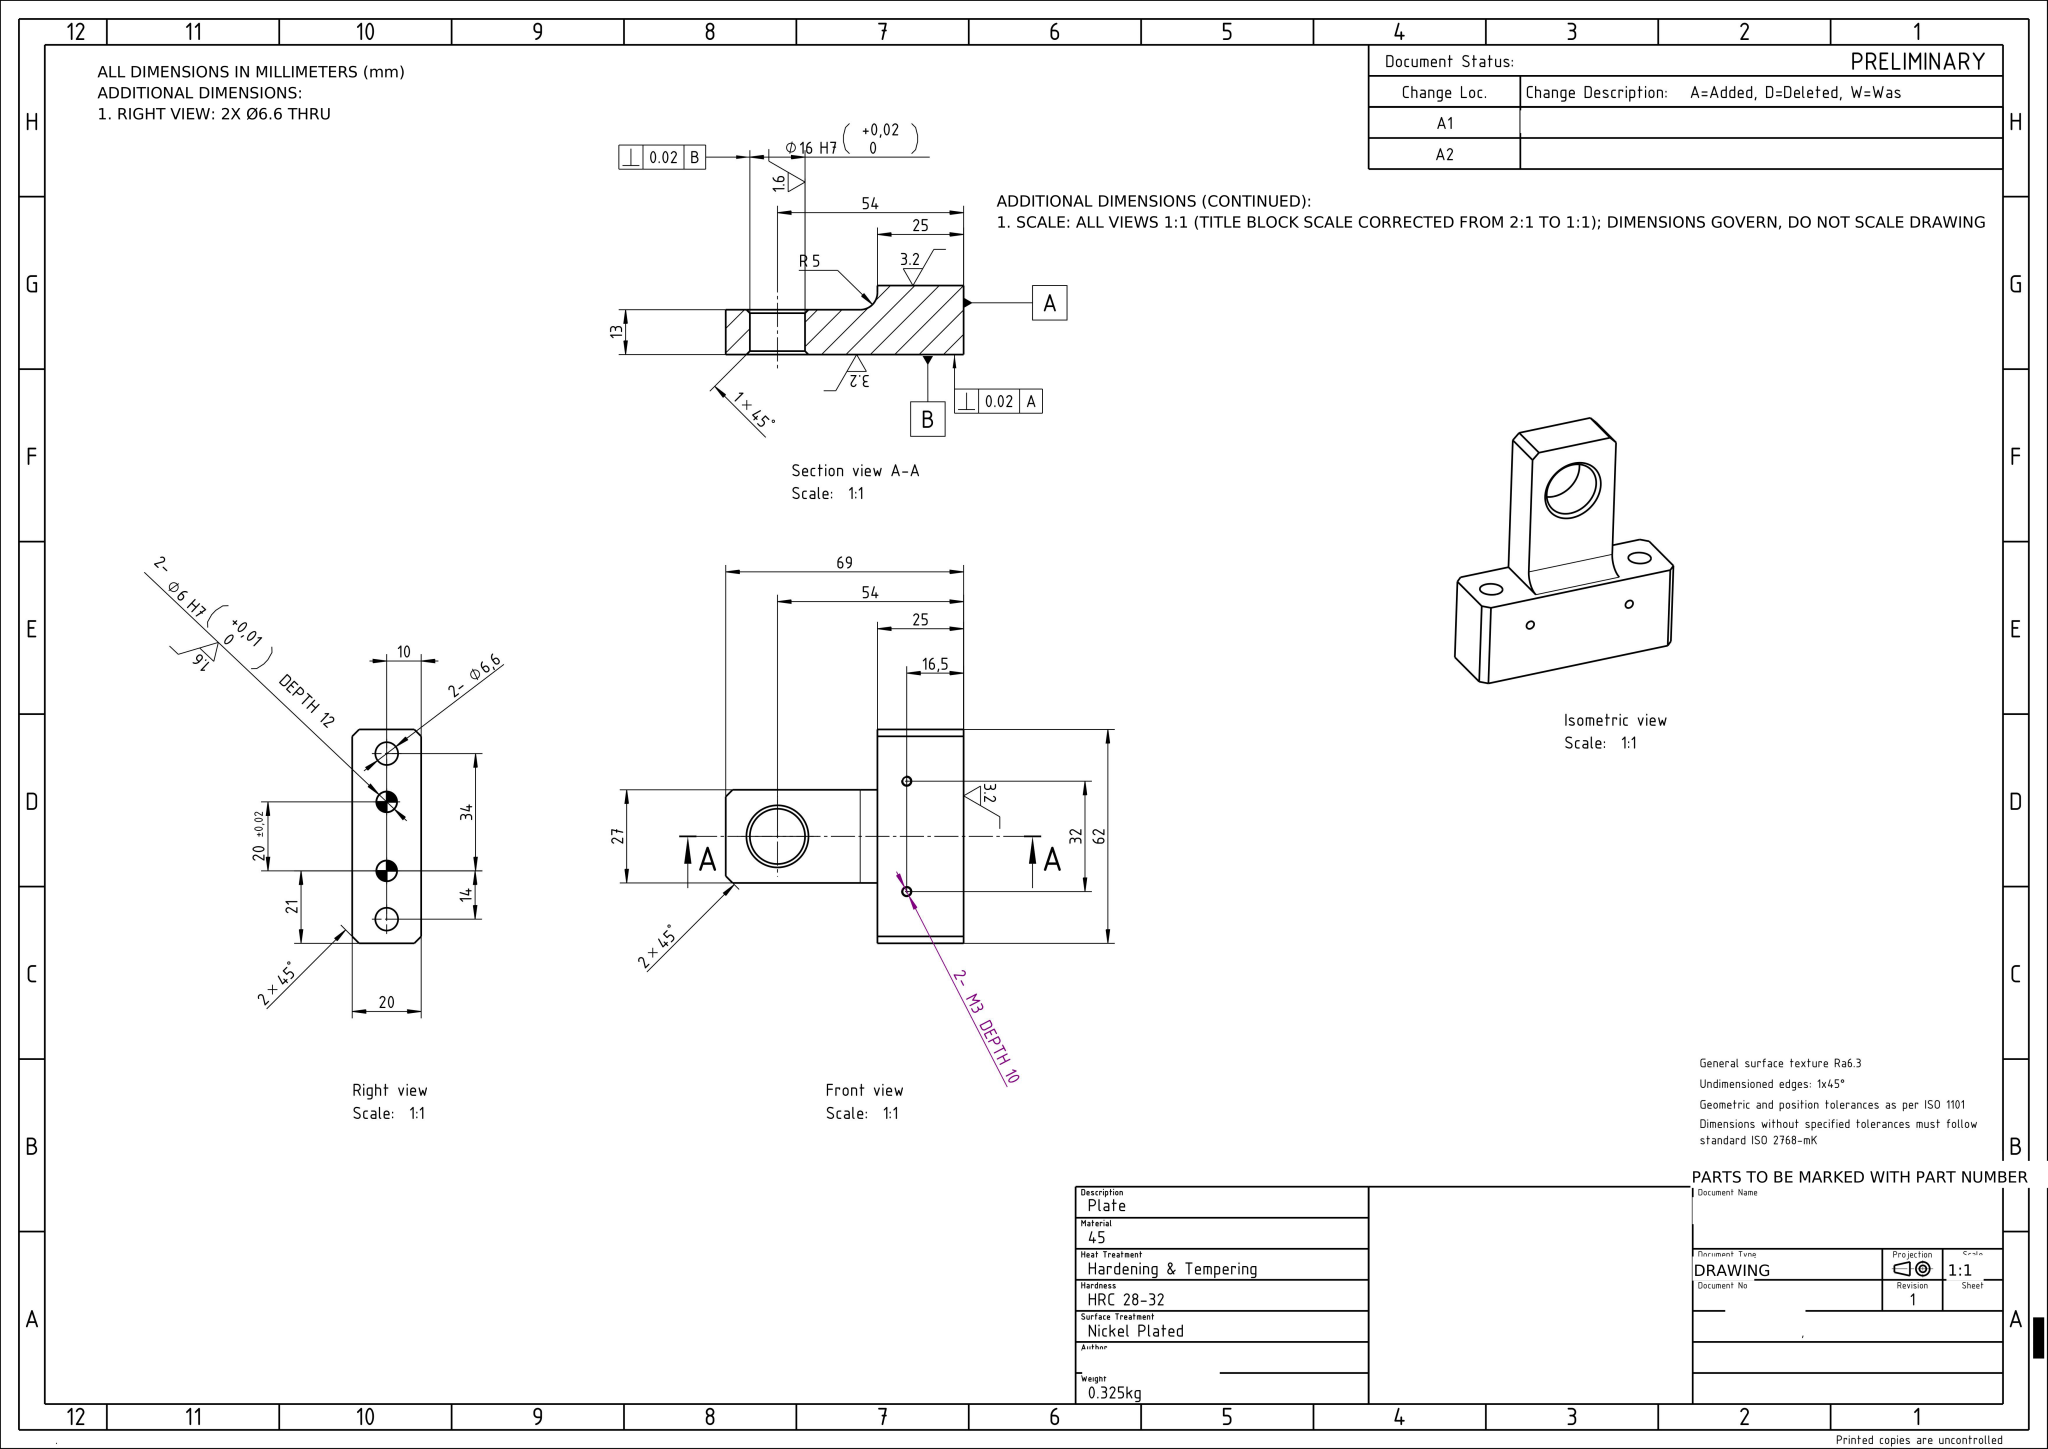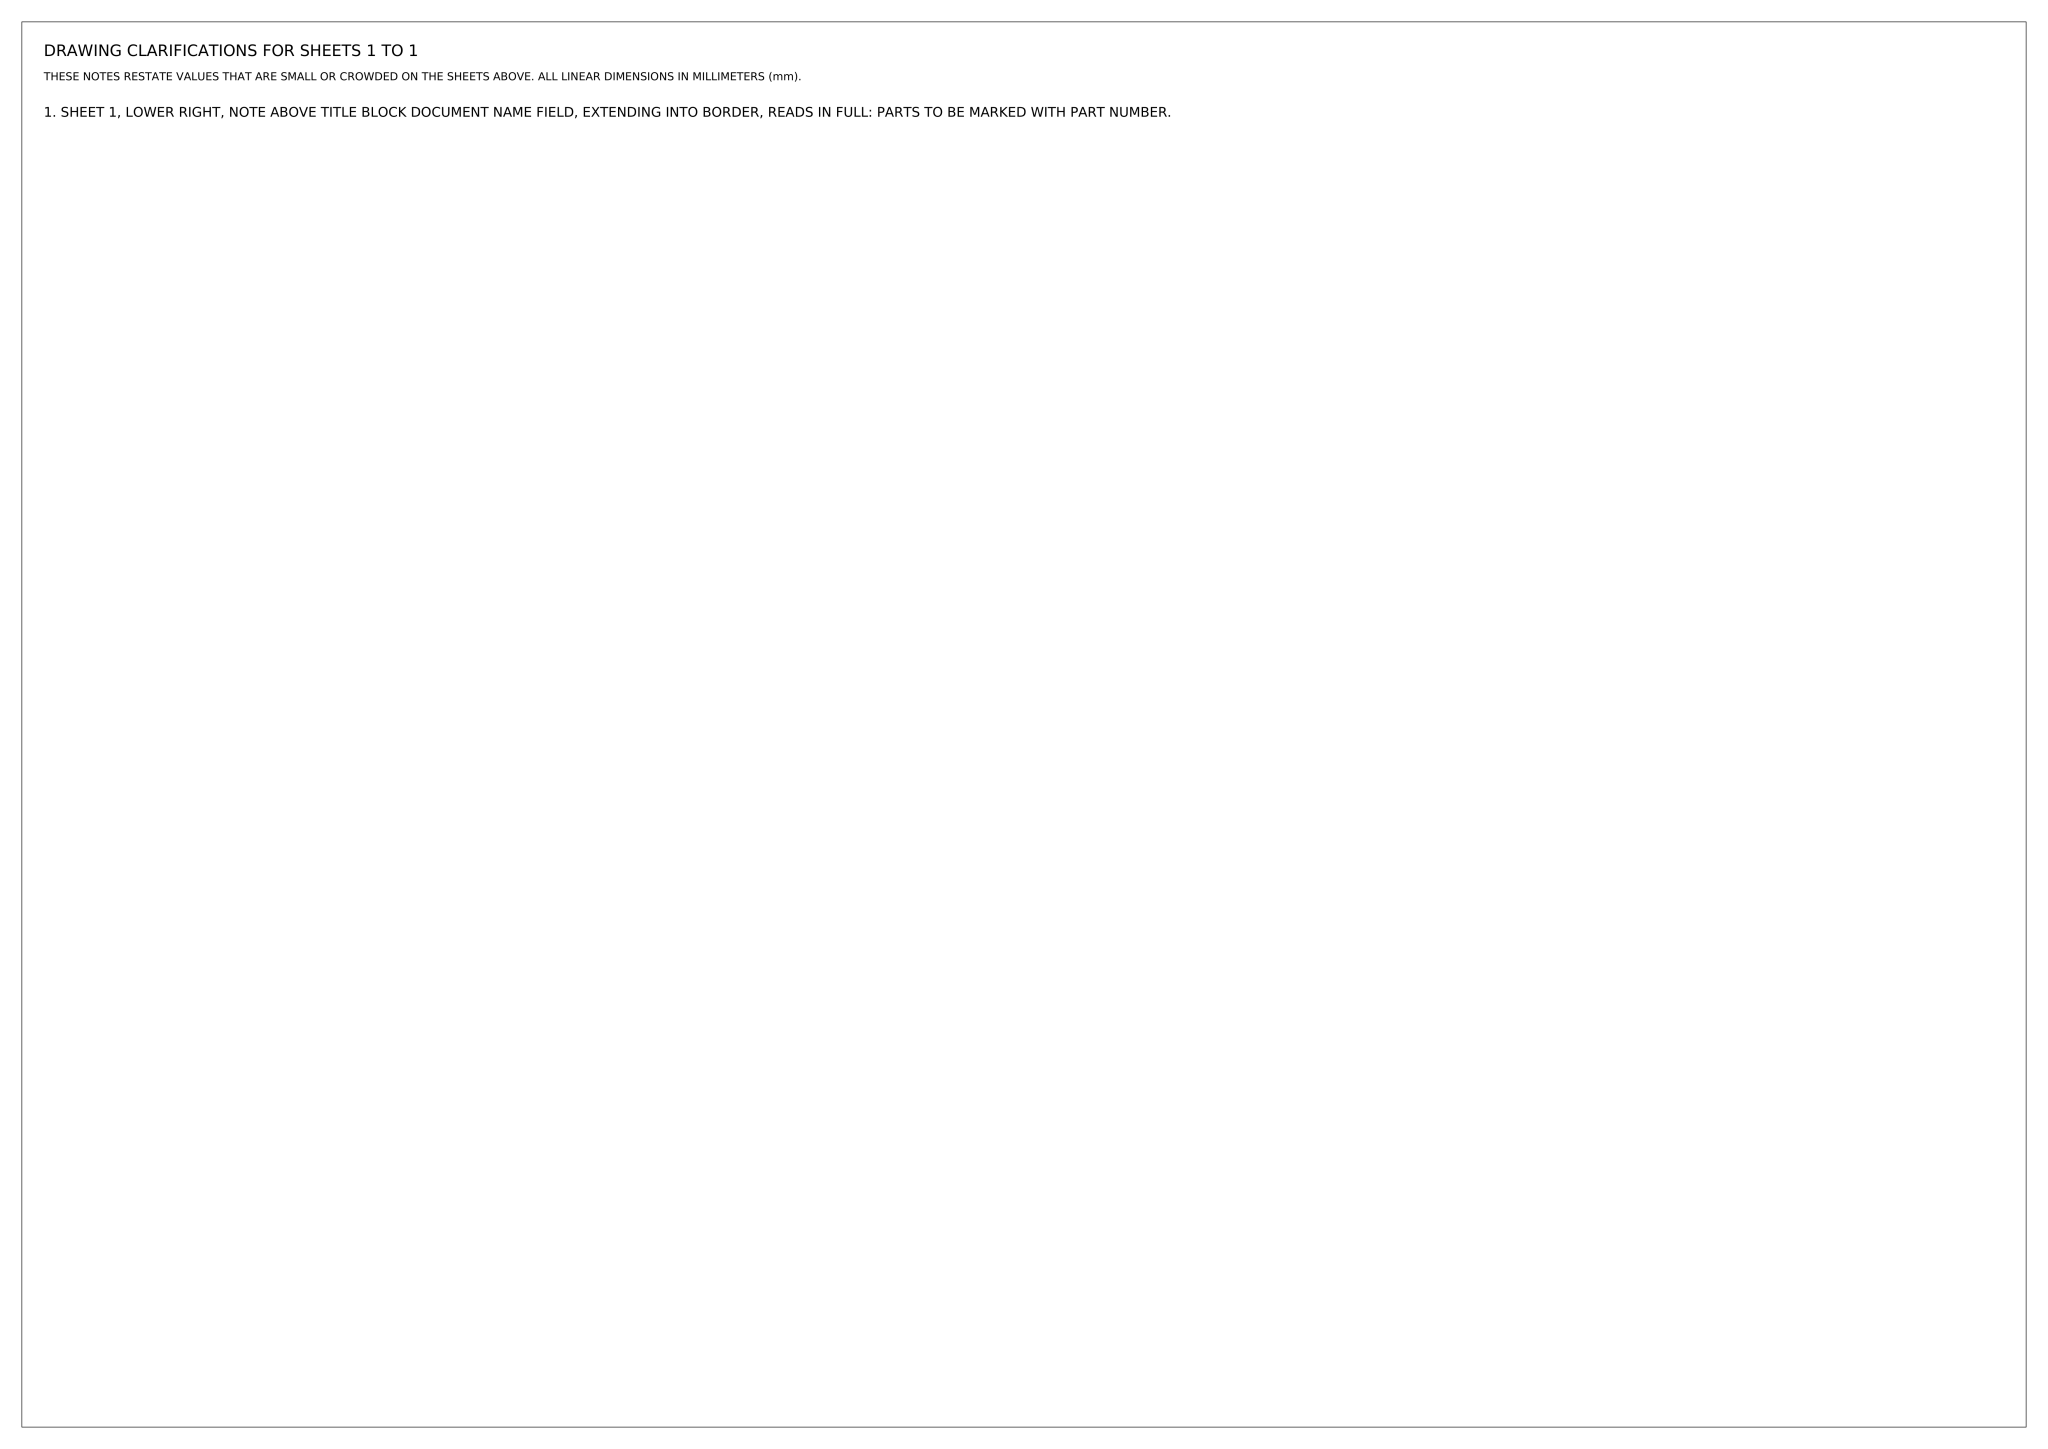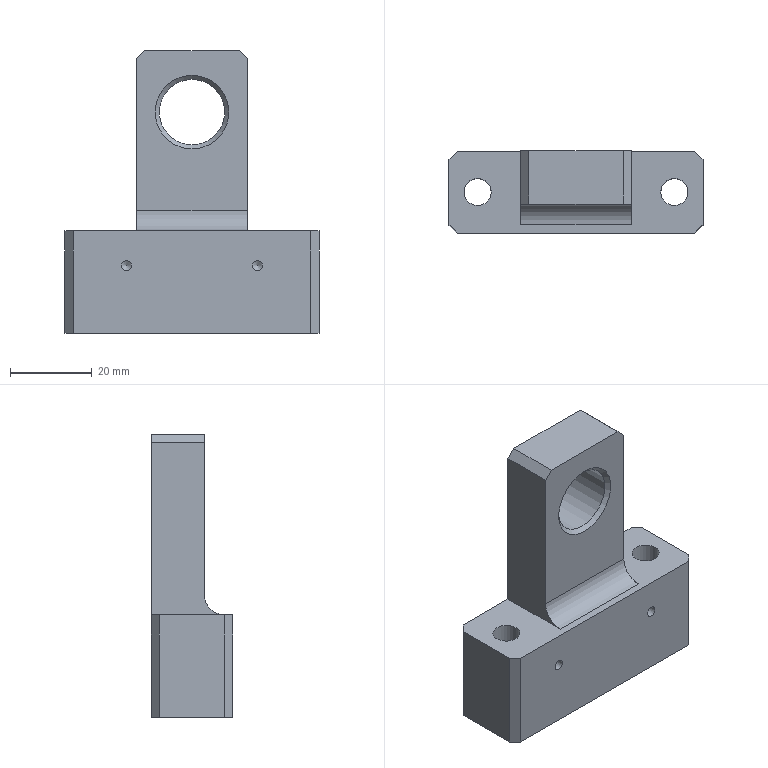Part | NX | mm | 1 solid | 30 faces | box 62 x 20 x 69 mm | volume 41127 mm3 | plane 16 | cylinder 8 | cone 6 | commonest cylinder face diameters 2.5 x2 6 x2 6.6 x2 10 x1 16 x1
STEP:
#1=CARTESIAN_POINT('',(0.,0.,0.));
#2=DIRECTION('',(0.,0.,1.));
#3=DIRECTION('',(1.,0.,0.));
#4=AXIS2_PLACEMENT_3D('',#1,#2,#3);
#5=(LENGTH_UNIT()NAMED_UNIT(*)SI_UNIT(.MILLI.,.METRE.));
#6=UNCERTAINTY_MEASURE_WITH_UNIT(LENGTH_MEASURE(0.00002),#5,'','');
#7=(NAMED_UNIT(*)PLANE_ANGLE_UNIT()SI_UNIT($,.RADIAN.));
#8=PLANE_ANGLE_MEASURE_WITH_UNIT(PLANE_ANGLE_MEASURE(0.01745),#7);
#9=DIMENSIONAL_EXPONENTS(0.,0.,0.,0.,0.,0.,0.);
#10=(CONVERSION_BASED_UNIT('',#8)NAMED_UNIT(#9)PLANE_ANGLE_UNIT());
#11=(NAMED_UNIT(*)SI_UNIT($,.STERADIAN.)SOLID_ANGLE_UNIT());
#12=(GEOMETRIC_REPRESENTATION_CONTEXT(3)GLOBAL_UNCERTAINTY_ASSIGNED_CONTEXT((#6))GLOBAL_UNIT_ASSIGNED_CONTEXT((#5,#10,#11))REPRESENTATION_CONTEXT('',''));
#13=SHAPE_REPRESENTATION('',(#4),#12);
#14=CARTESIAN_POINT('',(-31.,8.,25.));
#15=VERTEX_POINT('',#14);
#16=CARTESIAN_POINT('',(-31.,-8.,25.));
#17=VERTEX_POINT('',#16);
#18=CARTESIAN_POINT('',(-31.,10.,25.));
#19=DIRECTION('',(0.,-1.,0.));
#20=VECTOR('',#19,1.);
#21=LINE('',#18,#20);
#22=EDGE_CURVE('',#15,#17,#21,.T.);
#23=ORIENTED_EDGE('',*,*,#22,.F.);
#24=CARTESIAN_POINT('',(-31.,8.,0.));
#25=VERTEX_POINT('',#24);
#26=CARTESIAN_POINT('',(-31.,8.,25.));
#27=DIRECTION('',(0.,0.,-1.));
#28=VECTOR('',#27,1.);
#29=LINE('',#26,#28);
#30=EDGE_CURVE('',#15,#25,#29,.T.);
#31=ORIENTED_EDGE('',*,*,#30,.T.);
#32=CARTESIAN_POINT('',(-31.,-8.,0.));
#33=VERTEX_POINT('',#32);
#34=CARTESIAN_POINT('',(-31.,10.,0.));
#35=DIRECTION('',(0.,-1.,0.));
#36=VECTOR('',#35,1.);
#37=LINE('',#34,#36);
#38=EDGE_CURVE('',#25,#33,#37,.T.);
#39=ORIENTED_EDGE('',*,*,#38,.T.);
#40=CARTESIAN_POINT('',(-31.,-8.,25.));
#41=DIRECTION('',(0.,0.,1.));
#42=VECTOR('',#41,1.);
#43=LINE('',#40,#42);
#44=EDGE_CURVE('',#33,#17,#43,.T.);
#45=ORIENTED_EDGE('',*,*,#44,.T.);
#46=EDGE_LOOP('',(#23,#31,#39,#45));
#47=FACE_OUTER_BOUND('',#46,.T.);
#48=CARTESIAN_POINT('',(-31.,10.,25.));
#49=DIRECTION('',(1.,0.,0.));
#50=DIRECTION('',(-0.,1.,0.));
#51=AXIS2_PLACEMENT_3D('',#48,#49,#50);
#52=PLANE('',#51);
#53=ADVANCED_FACE('',(#47),#52,.F.);
#54=CARTESIAN_POINT('',(16.,-10.,17.75));
#55=VERTEX_POINT('',#54);
#56=CARTESIAN_POINT('',(16.,-10.,16.5));
#57=DIRECTION('',(0.,1.,0.));
#58=DIRECTION('',(0.,0.,1.));
#59=AXIS2_PLACEMENT_3D('',#56,#57,#58);
#60=CIRCLE('',#59,1.25);
#61=EDGE_CURVE('',#55,#55,#60,.T.);
#62=ORIENTED_EDGE('',*,*,#61,.T.);
#63=EDGE_LOOP('',(#62));
#64=FACE_BOUND('',#63,.T.);
#65=CARTESIAN_POINT('',(-16.,-10.,17.75));
#66=VERTEX_POINT('',#65);
#67=CARTESIAN_POINT('',(-16.,-10.,16.5));
#68=DIRECTION('',(0.,1.,0.));
#69=DIRECTION('',(0.,0.,1.));
#70=AXIS2_PLACEMENT_3D('',#67,#68,#69);
#71=CIRCLE('',#70,1.25);
#72=EDGE_CURVE('',#66,#66,#71,.T.);
#73=ORIENTED_EDGE('',*,*,#72,.T.);
#74=EDGE_LOOP('',(#73));
#75=FACE_BOUND('',#74,.T.);
#76=CARTESIAN_POINT('',(-29.,-10.,0.));
#77=VERTEX_POINT('',#76);
#78=CARTESIAN_POINT('',(29.,-10.,0.));
#79=VERTEX_POINT('',#78);
#80=CARTESIAN_POINT('',(-31.,-10.,0.));
#81=DIRECTION('',(1.,0.,0.));
#82=VECTOR('',#81,1.);
#83=LINE('',#80,#82);
#84=EDGE_CURVE('',#77,#79,#83,.T.);
#85=ORIENTED_EDGE('',*,*,#84,.T.);
#86=CARTESIAN_POINT('',(29.,-10.,25.));
#87=VERTEX_POINT('',#86);
#88=CARTESIAN_POINT('',(29.,-10.,25.));
#89=DIRECTION('',(0.,0.,1.));
#90=VECTOR('',#89,1.);
#91=LINE('',#88,#90);
#92=EDGE_CURVE('',#79,#87,#91,.T.);
#93=ORIENTED_EDGE('',*,*,#92,.T.);
#94=CARTESIAN_POINT('',(-29.,-10.,25.));
#95=VERTEX_POINT('',#94);
#96=CARTESIAN_POINT('',(-31.,-10.,25.));
#97=DIRECTION('',(1.,0.,0.));
#98=VECTOR('',#97,1.);
#99=LINE('',#96,#98);
#100=EDGE_CURVE('',#95,#87,#99,.T.);
#101=ORIENTED_EDGE('',*,*,#100,.F.);
#102=CARTESIAN_POINT('',(-29.,-10.,25.));
#103=DIRECTION('',(0.,0.,-1.));
#104=VECTOR('',#103,1.);
#105=LINE('',#102,#104);
#106=EDGE_CURVE('',#95,#77,#105,.T.);
#107=ORIENTED_EDGE('',*,*,#106,.T.);
#108=EDGE_LOOP('',(#85,#93,#101,#107));
#109=FACE_BOUND('',#108,.T.);
#110=CARTESIAN_POINT('',(-31.,-10.,25.));
#111=DIRECTION('',(0.,1.,0.));
#112=DIRECTION('',(0.,0.,1.));
#113=AXIS2_PLACEMENT_3D('',#110,#111,#112);
#114=PLANE('',#113);
#115=ADVANCED_FACE('',(#64,#75,#109),#114,.F.);
#116=CARTESIAN_POINT('',(31.,-8.,25.));
#117=VERTEX_POINT('',#116);
#118=CARTESIAN_POINT('',(31.,8.,25.));
#119=VERTEX_POINT('',#118);
#120=CARTESIAN_POINT('',(31.,-10.,25.));
#121=DIRECTION('',(-0.,1.,0.));
#122=VECTOR('',#121,1.);
#123=LINE('',#120,#122);
#124=EDGE_CURVE('',#117,#119,#123,.T.);
#125=ORIENTED_EDGE('',*,*,#124,.F.);
#126=CARTESIAN_POINT('',(31.,-8.,0.));
#127=VERTEX_POINT('',#126);
#128=CARTESIAN_POINT('',(31.,-8.,25.));
#129=DIRECTION('',(0.,0.,-1.));
#130=VECTOR('',#129,1.);
#131=LINE('',#128,#130);
#132=EDGE_CURVE('',#117,#127,#131,.T.);
#133=ORIENTED_EDGE('',*,*,#132,.T.);
#134=CARTESIAN_POINT('',(31.,8.,0.));
#135=VERTEX_POINT('',#134);
#136=CARTESIAN_POINT('',(31.,-10.,0.));
#137=DIRECTION('',(-0.,1.,0.));
#138=VECTOR('',#137,1.);
#139=LINE('',#136,#138);
#140=EDGE_CURVE('',#127,#135,#139,.T.);
#141=ORIENTED_EDGE('',*,*,#140,.T.);
#142=CARTESIAN_POINT('',(31.,8.,25.));
#143=DIRECTION('',(0.,0.,1.));
#144=VECTOR('',#143,1.);
#145=LINE('',#142,#144);
#146=EDGE_CURVE('',#135,#119,#145,.T.);
#147=ORIENTED_EDGE('',*,*,#146,.T.);
#148=EDGE_LOOP('',(#125,#133,#141,#147));
#149=FACE_OUTER_BOUND('',#148,.T.);
#150=CARTESIAN_POINT('',(31.,-10.,25.));
#151=DIRECTION('',(-1.,-0.,0.));
#152=DIRECTION('',(0.,-1.,0.));
#153=AXIS2_PLACEMENT_3D('',#150,#151,#152);
#154=PLANE('',#153);
#155=ADVANCED_FACE('',(#149),#154,.F.);
#156=CARTESIAN_POINT('',(0.,10.,45.));
#157=VERTEX_POINT('',#156);
#158=CARTESIAN_POINT('',(0.,10.,54.));
#159=DIRECTION('',(0.,-1.,0.));
#160=DIRECTION('',(0.,0.,-1.));
#161=AXIS2_PLACEMENT_3D('',#158,#159,#160);
#162=CIRCLE('',#161,9.);
#163=EDGE_CURVE('',#157,#157,#162,.T.);
#164=ORIENTED_EDGE('',*,*,#163,.T.);
#165=EDGE_LOOP('',(#164));
#166=FACE_BOUND('',#165,.T.);
#167=CARTESIAN_POINT('',(29.,10.,25.));
#168=VERTEX_POINT('',#167);
#169=CARTESIAN_POINT('',(13.5,10.,25.));
#170=VERTEX_POINT('',#169);
#171=CARTESIAN_POINT('',(31.,10.,25.));
#172=DIRECTION('',(-1.,0.,0.));
#173=VECTOR('',#172,1.);
#174=LINE('',#171,#173);
#175=EDGE_CURVE('',#168,#170,#174,.T.);
#176=ORIENTED_EDGE('',*,*,#175,.F.);
#177=CARTESIAN_POINT('',(29.,10.,0.));
#178=VERTEX_POINT('',#177);
#179=CARTESIAN_POINT('',(29.,10.,25.));
#180=DIRECTION('',(0.,0.,-1.));
#181=VECTOR('',#180,1.);
#182=LINE('',#179,#181);
#183=EDGE_CURVE('',#168,#178,#182,.T.);
#184=ORIENTED_EDGE('',*,*,#183,.T.);
#185=CARTESIAN_POINT('',(-29.,10.,0.));
#186=VERTEX_POINT('',#185);
#187=CARTESIAN_POINT('',(31.,10.,0.));
#188=DIRECTION('',(-1.,0.,0.));
#189=VECTOR('',#188,1.);
#190=LINE('',#187,#189);
#191=EDGE_CURVE('',#178,#186,#190,.T.);
#192=ORIENTED_EDGE('',*,*,#191,.T.);
#193=CARTESIAN_POINT('',(-29.,10.,25.));
#194=VERTEX_POINT('',#193);
#195=CARTESIAN_POINT('',(-29.,10.,25.));
#196=DIRECTION('',(0.,0.,1.));
#197=VECTOR('',#196,1.);
#198=LINE('',#195,#197);
#199=EDGE_CURVE('',#186,#194,#198,.T.);
#200=ORIENTED_EDGE('',*,*,#199,.T.);
#201=CARTESIAN_POINT('',(-13.5,10.,25.));
#202=VERTEX_POINT('',#201);
#203=CARTESIAN_POINT('',(31.,10.,25.));
#204=DIRECTION('',(-1.,0.,0.));
#205=VECTOR('',#204,1.);
#206=LINE('',#203,#205);
#207=EDGE_CURVE('',#202,#194,#206,.T.);
#208=ORIENTED_EDGE('',*,*,#207,.F.);
#209=CARTESIAN_POINT('',(-13.5,10.,67.));
#210=VERTEX_POINT('',#209);
#211=CARTESIAN_POINT('',(-13.5,10.,25.));
#212=DIRECTION('',(0.,0.,1.));
#213=VECTOR('',#212,1.);
#214=LINE('',#211,#213);
#215=EDGE_CURVE('',#202,#210,#214,.T.);
#216=ORIENTED_EDGE('',*,*,#215,.T.);
#217=CARTESIAN_POINT('',(-11.5,10.,69.));
#218=VERTEX_POINT('',#217);
#219=CARTESIAN_POINT('',(-13.5,10.,67.));
#220=DIRECTION('',(0.7071,0.,0.7071));
#221=VECTOR('',#220,1.);
#222=LINE('',#219,#221);
#223=EDGE_CURVE('',#210,#218,#222,.T.);
#224=ORIENTED_EDGE('',*,*,#223,.T.);
#225=CARTESIAN_POINT('',(11.5,10.,69.));
#226=VERTEX_POINT('',#225);
#227=CARTESIAN_POINT('',(-13.5,10.,69.));
#228=DIRECTION('',(1.,0.,0.));
#229=VECTOR('',#228,1.);
#230=LINE('',#227,#229);
#231=EDGE_CURVE('',#218,#226,#230,.T.);
#232=ORIENTED_EDGE('',*,*,#231,.T.);
#233=CARTESIAN_POINT('',(13.5,10.,67.));
#234=VERTEX_POINT('',#233);
#235=CARTESIAN_POINT('',(11.5,10.,69.));
#236=DIRECTION('',(0.7071,0.,-0.7071));
#237=VECTOR('',#236,1.);
#238=LINE('',#235,#237);
#239=EDGE_CURVE('',#226,#234,#238,.T.);
#240=ORIENTED_EDGE('',*,*,#239,.T.);
#241=CARTESIAN_POINT('',(13.5,10.,69.));
#242=DIRECTION('',(0.,0.,-1.));
#243=VECTOR('',#242,1.);
#244=LINE('',#241,#243);
#245=EDGE_CURVE('',#234,#170,#244,.T.);
#246=ORIENTED_EDGE('',*,*,#245,.T.);
#247=EDGE_LOOP('',(#176,#184,#192,#200,#208,#216,#224,#232,#240,#246));
#248=FACE_BOUND('',#247,.T.);
#249=CARTESIAN_POINT('',(31.,10.,25.));
#250=DIRECTION('',(0.,-1.,0.));
#251=DIRECTION('',(0.,0.,-1.));
#252=AXIS2_PLACEMENT_3D('',#249,#250,#251);
#253=PLANE('',#252);
#254=ADVANCED_FACE('',(#166,#248),#253,.F.);
#255=CARTESIAN_POINT('',(27.3,0.,25.));
#256=VERTEX_POINT('',#255);
#257=CARTESIAN_POINT('',(24.,0.,25.));
#258=DIRECTION('',(0.,0.,1.));
#259=DIRECTION('',(1.,0.,0.));
#260=AXIS2_PLACEMENT_3D('',#257,#258,#259);
#261=CIRCLE('',#260,3.3);
#262=EDGE_CURVE('',#256,#256,#261,.T.);
#263=ORIENTED_EDGE('',*,*,#262,.F.);
#264=EDGE_LOOP('',(#263));
#265=FACE_BOUND('',#264,.T.);
#266=CARTESIAN_POINT('',(-20.7,0.,25.));
#267=VERTEX_POINT('',#266);
#268=CARTESIAN_POINT('',(-24.,0.,25.));
#269=DIRECTION('',(0.,0.,1.));
#270=DIRECTION('',(1.,0.,0.));
#271=AXIS2_PLACEMENT_3D('',#268,#269,#270);
#272=CIRCLE('',#271,3.3);
#273=EDGE_CURVE('',#267,#267,#272,.T.);
#274=ORIENTED_EDGE('',*,*,#273,.F.);
#275=EDGE_LOOP('',(#274));
#276=FACE_BOUND('',#275,.T.);
#277=ORIENTED_EDGE('',*,*,#100,.T.);
#278=CARTESIAN_POINT('',(19.5,-19.5,25.));
#279=DIRECTION('',(0.7071,0.7071,0.));
#280=VECTOR('',#279,1.);
#281=LINE('',#278,#280);
#282=EDGE_CURVE('',#87,#117,#281,.T.);
#283=ORIENTED_EDGE('',*,*,#282,.T.);
#284=ORIENTED_EDGE('',*,*,#124,.T.);
#285=CARTESIAN_POINT('',(19.5,19.5,25.));
#286=DIRECTION('',(-0.7071,0.7071,0.));
#287=VECTOR('',#286,1.);
#288=LINE('',#285,#287);
#289=EDGE_CURVE('',#119,#168,#288,.T.);
#290=ORIENTED_EDGE('',*,*,#289,.T.);
#291=ORIENTED_EDGE('',*,*,#175,.T.);
#292=CARTESIAN_POINT('',(13.5,-8.,25.));
#293=VERTEX_POINT('',#292);
#294=CARTESIAN_POINT('',(13.5,-3.,25.));
#295=DIRECTION('',(0.,1.,0.));
#296=VECTOR('',#295,1.);
#297=LINE('',#294,#296);
#298=EDGE_CURVE('',#293,#170,#297,.T.);
#299=ORIENTED_EDGE('',*,*,#298,.F.);
#300=CARTESIAN_POINT('',(-13.5,-8.,25.));
#301=VERTEX_POINT('',#300);
#302=CARTESIAN_POINT('',(0.,-8.,25.));
#303=DIRECTION('',(-1.,0.,0.));
#304=VECTOR('',#303,1.);
#305=LINE('',#302,#304);
#306=EDGE_CURVE('',#293,#301,#305,.T.);
#307=ORIENTED_EDGE('',*,*,#306,.T.);
#308=CARTESIAN_POINT('',(-13.5,-3.,25.));
#309=DIRECTION('',(0.,1.,0.));
#310=VECTOR('',#309,1.);
#311=LINE('',#308,#310);
#312=EDGE_CURVE('',#301,#202,#311,.T.);
#313=ORIENTED_EDGE('',*,*,#312,.T.);
#314=ORIENTED_EDGE('',*,*,#207,.T.);
#315=CARTESIAN_POINT('',(-19.5,19.5,25.));
#316=DIRECTION('',(-0.7071,-0.7071,0.));
#317=VECTOR('',#316,1.);
#318=LINE('',#315,#317);
#319=EDGE_CURVE('',#194,#15,#318,.T.);
#320=ORIENTED_EDGE('',*,*,#319,.T.);
#321=ORIENTED_EDGE('',*,*,#22,.T.);
#322=CARTESIAN_POINT('',(-19.5,-19.5,25.));
#323=DIRECTION('',(0.7071,-0.7071,0.));
#324=VECTOR('',#323,1.);
#325=LINE('',#322,#324);
#326=EDGE_CURVE('',#17,#95,#325,.T.);
#327=ORIENTED_EDGE('',*,*,#326,.T.);
#328=EDGE_LOOP('',(#277,#283,#284,#290,#291,#299,#307,#313,#314,#320,#321,#327));
#329=FACE_BOUND('',#328,.T.);
#330=CARTESIAN_POINT('',(0.,0.,25.));
#331=DIRECTION('',(0.,0.,1.));
#332=DIRECTION('',(1.,0.,0.));
#333=AXIS2_PLACEMENT_3D('',#330,#331,#332);
#334=PLANE('',#333);
#335=ADVANCED_FACE('',(#265,#276,#329),#334,.T.);
#336=CARTESIAN_POINT('',(27.3,0.,0.));
#337=VERTEX_POINT('',#336);
#338=CARTESIAN_POINT('',(24.,0.,0.));
#339=DIRECTION('',(0.,0.,1.));
#340=DIRECTION('',(1.,0.,0.));
#341=AXIS2_PLACEMENT_3D('',#338,#339,#340);
#342=CIRCLE('',#341,3.3);
#343=EDGE_CURVE('',#337,#337,#342,.T.);
#344=ORIENTED_EDGE('',*,*,#343,.T.);
#345=EDGE_LOOP('',(#344));
#346=FACE_BOUND('',#345,.T.);
#347=CARTESIAN_POINT('',(-20.7,0.,0.));
#348=VERTEX_POINT('',#347);
#349=CARTESIAN_POINT('',(-24.,0.,0.));
#350=DIRECTION('',(0.,0.,1.));
#351=DIRECTION('',(1.,0.,0.));
#352=AXIS2_PLACEMENT_3D('',#349,#350,#351);
#353=CIRCLE('',#352,3.3);
#354=EDGE_CURVE('',#348,#348,#353,.T.);
#355=ORIENTED_EDGE('',*,*,#354,.T.);
#356=EDGE_LOOP('',(#355));
#357=FACE_BOUND('',#356,.T.);
#358=CARTESIAN_POINT('',(13.,0.,0.));
#359=VERTEX_POINT('',#358);
#360=CARTESIAN_POINT('',(10.,0.,0.));
#361=DIRECTION('',(0.,0.,1.));
#362=DIRECTION('',(1.,0.,0.));
#363=AXIS2_PLACEMENT_3D('',#360,#361,#362);
#364=CIRCLE('',#363,3.);
#365=EDGE_CURVE('',#359,#359,#364,.T.);
#366=ORIENTED_EDGE('',*,*,#365,.T.);
#367=EDGE_LOOP('',(#366));
#368=FACE_BOUND('',#367,.T.);
#369=CARTESIAN_POINT('',(-7.,0.,0.));
#370=VERTEX_POINT('',#369);
#371=CARTESIAN_POINT('',(-10.,0.,0.));
#372=DIRECTION('',(0.,0.,1.));
#373=DIRECTION('',(1.,0.,0.));
#374=AXIS2_PLACEMENT_3D('',#371,#372,#373);
#375=CIRCLE('',#374,3.);
#376=EDGE_CURVE('',#370,#370,#375,.T.);
#377=ORIENTED_EDGE('',*,*,#376,.T.);
#378=EDGE_LOOP('',(#377));
#379=FACE_BOUND('',#378,.T.);
#380=ORIENTED_EDGE('',*,*,#140,.F.);
#381=CARTESIAN_POINT('',(31.,-8.,0.));
#382=DIRECTION('',(-0.7071,-0.7071,0.));
#383=VECTOR('',#382,1.);
#384=LINE('',#381,#383);
#385=EDGE_CURVE('',#127,#79,#384,.T.);
#386=ORIENTED_EDGE('',*,*,#385,.T.);
#387=ORIENTED_EDGE('',*,*,#84,.F.);
#388=CARTESIAN_POINT('',(-29.,-10.,0.));
#389=DIRECTION('',(-0.7071,0.7071,0.));
#390=VECTOR('',#389,1.);
#391=LINE('',#388,#390);
#392=EDGE_CURVE('',#77,#33,#391,.T.);
#393=ORIENTED_EDGE('',*,*,#392,.T.);
#394=ORIENTED_EDGE('',*,*,#38,.F.);
#395=CARTESIAN_POINT('',(-31.,8.,0.));
#396=DIRECTION('',(0.7071,0.7071,0.));
#397=VECTOR('',#396,1.);
#398=LINE('',#395,#397);
#399=EDGE_CURVE('',#25,#186,#398,.T.);
#400=ORIENTED_EDGE('',*,*,#399,.T.);
#401=ORIENTED_EDGE('',*,*,#191,.F.);
#402=CARTESIAN_POINT('',(29.,10.,0.));
#403=DIRECTION('',(0.7071,-0.7071,0.));
#404=VECTOR('',#403,1.);
#405=LINE('',#402,#404);
#406=EDGE_CURVE('',#178,#135,#405,.T.);
#407=ORIENTED_EDGE('',*,*,#406,.T.);
#408=EDGE_LOOP('',(#380,#386,#387,#393,#394,#400,#401,#407));
#409=FACE_BOUND('',#408,.T.);
#410=CARTESIAN_POINT('',(0.,0.,0.));
#411=DIRECTION('',(0.,0.,1.));
#412=DIRECTION('',(1.,0.,0.));
#413=AXIS2_PLACEMENT_3D('',#410,#411,#412);
#414=PLANE('',#413);
#415=ADVANCED_FACE('',(#346,#357,#368,#379,#409),#414,.F.);
#416=CARTESIAN_POINT('',(-13.5,-3.,30.));
#417=VERTEX_POINT('',#416);
#418=CARTESIAN_POINT('',(-13.5,-3.,67.));
#419=VERTEX_POINT('',#418);
#420=CARTESIAN_POINT('',(-13.5,-3.,25.));
#421=DIRECTION('',(0.,0.,1.));
#422=VECTOR('',#421,1.);
#423=LINE('',#420,#422);
#424=EDGE_CURVE('',#417,#419,#423,.T.);
#425=ORIENTED_EDGE('',*,*,#424,.T.);
#426=CARTESIAN_POINT('',(-13.5,-3.,67.));
#427=DIRECTION('',(0.,1.,0.));
#428=VECTOR('',#427,1.);
#429=LINE('',#426,#428);
#430=EDGE_CURVE('',#419,#210,#429,.T.);
#431=ORIENTED_EDGE('',*,*,#430,.T.);
#432=ORIENTED_EDGE('',*,*,#215,.F.);
#433=ORIENTED_EDGE('',*,*,#312,.F.);
#434=CARTESIAN_POINT('',(-13.5,-8.,30.));
#435=DIRECTION('',(1.,0.,0.));
#436=DIRECTION('',(0.,0.,1.));
#437=AXIS2_PLACEMENT_3D('',#434,#435,#436);
#438=CIRCLE('',#437,5.);
#439=EDGE_CURVE('',#301,#417,#438,.T.);
#440=ORIENTED_EDGE('',*,*,#439,.T.);
#441=EDGE_LOOP('',(#425,#431,#432,#433,#440));
#442=FACE_OUTER_BOUND('',#441,.T.);
#443=CARTESIAN_POINT('',(-13.5,-3.,25.));
#444=DIRECTION('',(-1.,0.,0.));
#445=DIRECTION('',(0.,0.,1.));
#446=AXIS2_PLACEMENT_3D('',#443,#444,#445);
#447=PLANE('',#446);
#448=ADVANCED_FACE('',(#442),#447,.T.);
#449=ORIENTED_EDGE('',*,*,#231,.F.);
#450=CARTESIAN_POINT('',(-11.5,-3.,69.));
#451=VERTEX_POINT('',#450);
#452=CARTESIAN_POINT('',(-11.5,-3.,69.));
#453=DIRECTION('',(0.,-1.,0.));
#454=VECTOR('',#453,1.);
#455=LINE('',#452,#454);
#456=EDGE_CURVE('',#218,#451,#455,.T.);
#457=ORIENTED_EDGE('',*,*,#456,.T.);
#458=CARTESIAN_POINT('',(11.5,-3.,69.));
#459=VERTEX_POINT('',#458);
#460=CARTESIAN_POINT('',(-13.5,-3.,69.));
#461=DIRECTION('',(1.,0.,0.));
#462=VECTOR('',#461,1.);
#463=LINE('',#460,#462);
#464=EDGE_CURVE('',#451,#459,#463,.T.);
#465=ORIENTED_EDGE('',*,*,#464,.T.);
#466=CARTESIAN_POINT('',(11.5,-3.,69.));
#467=DIRECTION('',(0.,1.,0.));
#468=VECTOR('',#467,1.);
#469=LINE('',#466,#468);
#470=EDGE_CURVE('',#459,#226,#469,.T.);
#471=ORIENTED_EDGE('',*,*,#470,.T.);
#472=EDGE_LOOP('',(#449,#457,#465,#471));
#473=FACE_OUTER_BOUND('',#472,.T.);
#474=CARTESIAN_POINT('',(-13.5,-3.,69.));
#475=DIRECTION('',(0.,0.,1.));
#476=DIRECTION('',(1.,0.,0.));
#477=AXIS2_PLACEMENT_3D('',#474,#475,#476);
#478=PLANE('',#477);
#479=ADVANCED_FACE('',(#473),#478,.T.);
#480=ORIENTED_EDGE('',*,*,#245,.F.);
#481=CARTESIAN_POINT('',(13.5,-3.,67.));
#482=VERTEX_POINT('',#481);
#483=CARTESIAN_POINT('',(13.5,-3.,67.));
#484=DIRECTION('',(0.,-1.,0.));
#485=VECTOR('',#484,1.);
#486=LINE('',#483,#485);
#487=EDGE_CURVE('',#234,#482,#486,.T.);
#488=ORIENTED_EDGE('',*,*,#487,.T.);
#489=CARTESIAN_POINT('',(13.5,-3.,30.));
#490=VERTEX_POINT('',#489);
#491=CARTESIAN_POINT('',(13.5,-3.,69.));
#492=DIRECTION('',(0.,0.,-1.));
#493=VECTOR('',#492,1.);
#494=LINE('',#491,#493);
#495=EDGE_CURVE('',#482,#490,#494,.T.);
#496=ORIENTED_EDGE('',*,*,#495,.T.);
#497=CARTESIAN_POINT('',(13.5,-8.,30.));
#498=DIRECTION('',(-1.,0.,0.));
#499=DIRECTION('',(0.,0.,-1.));
#500=AXIS2_PLACEMENT_3D('',#497,#498,#499);
#501=CIRCLE('',#500,5.);
#502=EDGE_CURVE('',#490,#293,#501,.T.);
#503=ORIENTED_EDGE('',*,*,#502,.T.);
#504=ORIENTED_EDGE('',*,*,#298,.T.);
#505=EDGE_LOOP('',(#480,#488,#496,#503,#504));
#506=FACE_OUTER_BOUND('',#505,.T.);
#507=CARTESIAN_POINT('',(13.5,-3.,69.));
#508=DIRECTION('',(1.,0.,0.));
#509=DIRECTION('',(0.,0.,-1.));
#510=AXIS2_PLACEMENT_3D('',#507,#508,#509);
#511=PLANE('',#510);
#512=ADVANCED_FACE('',(#506),#511,.T.);
#513=CARTESIAN_POINT('',(0.,-3.,63.));
#514=VERTEX_POINT('',#513);
#515=CARTESIAN_POINT('',(0.,-3.,54.));
#516=DIRECTION('',(0.,1.,0.));
#517=DIRECTION('',(0.,0.,1.));
#518=AXIS2_PLACEMENT_3D('',#515,#516,#517);
#519=CIRCLE('',#518,9.);
#520=EDGE_CURVE('',#514,#514,#519,.T.);
#521=ORIENTED_EDGE('',*,*,#520,.T.);
#522=EDGE_LOOP('',(#521));
#523=FACE_BOUND('',#522,.T.);
#524=ORIENTED_EDGE('',*,*,#464,.F.);
#525=CARTESIAN_POINT('',(-13.5,-3.,67.));
#526=DIRECTION('',(-0.7071,0.,-0.7071));
#527=VECTOR('',#526,1.);
#528=LINE('',#525,#527);
#529=EDGE_CURVE('',#451,#419,#528,.T.);
#530=ORIENTED_EDGE('',*,*,#529,.T.);
#531=ORIENTED_EDGE('',*,*,#424,.F.);
#532=CARTESIAN_POINT('',(0.,-3.,30.));
#533=DIRECTION('',(1.,0.,0.));
#534=VECTOR('',#533,1.);
#535=LINE('',#532,#534);
#536=EDGE_CURVE('',#417,#490,#535,.T.);
#537=ORIENTED_EDGE('',*,*,#536,.T.);
#538=ORIENTED_EDGE('',*,*,#495,.F.);
#539=CARTESIAN_POINT('',(11.5,-3.,69.));
#540=DIRECTION('',(-0.7071,0.,0.7071));
#541=VECTOR('',#540,1.);
#542=LINE('',#539,#541);
#543=EDGE_CURVE('',#482,#459,#542,.T.);
#544=ORIENTED_EDGE('',*,*,#543,.T.);
#545=EDGE_LOOP('',(#524,#530,#531,#537,#538,#544));
#546=FACE_BOUND('',#545,.T.);
#547=CARTESIAN_POINT('',(0.,-3.,0.));
#548=DIRECTION('',(0.,1.,0.));
#549=DIRECTION('',(0.,0.,1.));
#550=AXIS2_PLACEMENT_3D('',#547,#548,#549);
#551=PLANE('',#550);
#552=ADVANCED_FACE('',(#523,#546),#551,.F.);
#553=ORIENTED_EDGE('',*,*,#502,.F.);
#554=ORIENTED_EDGE('',*,*,#536,.F.);
#555=ORIENTED_EDGE('',*,*,#439,.F.);
#556=ORIENTED_EDGE('',*,*,#306,.F.);
#557=EDGE_LOOP('',(#553,#554,#555,#556));
#558=FACE_OUTER_BOUND('',#557,.T.);
#559=CARTESIAN_POINT('',(0.,-8.,30.));
#560=DIRECTION('',(-1.,0.,0.));
#561=DIRECTION('',(0.,0.,1.));
#562=AXIS2_PLACEMENT_3D('',#559,#560,#561);
#563=CYLINDRICAL_SURFACE('',#562,5.);
#564=ADVANCED_FACE('',(#558),#563,.F.);
#565=CARTESIAN_POINT('',(-16.,2.,17.75));
#566=VERTEX_POINT('',#565);
#567=CARTESIAN_POINT('',(-16.,2.,16.5));
#568=DIRECTION('',(0.,-1.,0.));
#569=DIRECTION('',(0.,0.,1.));
#570=AXIS2_PLACEMENT_3D('',#567,#568,#569);
#571=CIRCLE('',#570,1.25);
#572=EDGE_CURVE('',#566,#566,#571,.T.);
#573=ORIENTED_EDGE('',*,*,#572,.T.);
#574=EDGE_LOOP('',(#573));
#575=FACE_BOUND('',#574,.T.);
#576=CARTESIAN_POINT('',(-16.,2.751,16.5));
#577=VERTEX_POINT('',#576);
#578=VERTEX_LOOP('',#577);
#579=FACE_BOUND('',#578,.T.);
#580=CARTESIAN_POINT('',(-16.,2.,16.5));
#581=DIRECTION('',(0.,-1.,0.));
#582=DIRECTION('',(0.,0.,-1.));
#583=AXIS2_PLACEMENT_3D('',#580,#581,#582);
#584=CONICAL_SURFACE('',#583,1.25,59.);
#585=ADVANCED_FACE('',(#575,#579),#584,.F.);
#586=ORIENTED_EDGE('',*,*,#572,.F.);
#587=EDGE_LOOP('',(#586));
#588=FACE_BOUND('',#587,.T.);
#589=ORIENTED_EDGE('',*,*,#72,.F.);
#590=EDGE_LOOP('',(#589));
#591=FACE_BOUND('',#590,.T.);
#592=CARTESIAN_POINT('',(-16.,-10.,16.5));
#593=DIRECTION('',(0.,1.,0.));
#594=DIRECTION('',(0.,0.,1.));
#595=AXIS2_PLACEMENT_3D('',#592,#593,#594);
#596=CYLINDRICAL_SURFACE('',#595,1.25);
#597=ADVANCED_FACE('',(#588,#591),#596,.F.);
#598=CARTESIAN_POINT('',(16.,2.,17.75));
#599=VERTEX_POINT('',#598);
#600=CARTESIAN_POINT('',(16.,2.,16.5));
#601=DIRECTION('',(0.,-1.,0.));
#602=DIRECTION('',(0.,0.,1.));
#603=AXIS2_PLACEMENT_3D('',#600,#601,#602);
#604=CIRCLE('',#603,1.25);
#605=EDGE_CURVE('',#599,#599,#604,.T.);
#606=ORIENTED_EDGE('',*,*,#605,.T.);
#607=EDGE_LOOP('',(#606));
#608=FACE_BOUND('',#607,.T.);
#609=CARTESIAN_POINT('',(16.,2.751,16.5));
#610=VERTEX_POINT('',#609);
#611=VERTEX_LOOP('',#610);
#612=FACE_BOUND('',#611,.T.);
#613=CARTESIAN_POINT('',(16.,2.,16.5));
#614=DIRECTION('',(0.,-1.,0.));
#615=DIRECTION('',(0.,0.,-1.));
#616=AXIS2_PLACEMENT_3D('',#613,#614,#615);
#617=CONICAL_SURFACE('',#616,1.25,59.);
#618=ADVANCED_FACE('',(#608,#612),#617,.F.);
#619=ORIENTED_EDGE('',*,*,#605,.F.);
#620=EDGE_LOOP('',(#619));
#621=FACE_BOUND('',#620,.T.);
#622=ORIENTED_EDGE('',*,*,#61,.F.);
#623=EDGE_LOOP('',(#622));
#624=FACE_BOUND('',#623,.T.);
#625=CARTESIAN_POINT('',(16.,-10.,16.5));
#626=DIRECTION('',(0.,1.,0.));
#627=DIRECTION('',(0.,0.,1.));
#628=AXIS2_PLACEMENT_3D('',#625,#626,#627);
#629=CYLINDRICAL_SURFACE('',#628,1.25);
#630=ADVANCED_FACE('',(#621,#624),#629,.F.);
#631=CARTESIAN_POINT('',(0.,9.,62.));
#632=VERTEX_POINT('',#631);
#633=CARTESIAN_POINT('',(0.,9.,54.));
#634=DIRECTION('',(0.,1.,0.));
#635=DIRECTION('',(0.,0.,1.));
#636=AXIS2_PLACEMENT_3D('',#633,#634,#635);
#637=CIRCLE('',#636,8.);
#638=EDGE_CURVE('',#632,#632,#637,.T.);
#639=ORIENTED_EDGE('',*,*,#638,.T.);
#640=EDGE_LOOP('',(#639));
#641=FACE_BOUND('',#640,.T.);
#642=CARTESIAN_POINT('',(0.,-2.,46.));
#643=VERTEX_POINT('',#642);
#644=CARTESIAN_POINT('',(0.,-2.,54.));
#645=DIRECTION('',(0.,-1.,0.));
#646=DIRECTION('',(0.,0.,-1.));
#647=AXIS2_PLACEMENT_3D('',#644,#645,#646);
#648=CIRCLE('',#647,8.);
#649=EDGE_CURVE('',#643,#643,#648,.T.);
#650=ORIENTED_EDGE('',*,*,#649,.T.);
#651=EDGE_LOOP('',(#650));
#652=FACE_BOUND('',#651,.T.);
#653=CARTESIAN_POINT('',(0.,-3.,54.));
#654=DIRECTION('',(0.,1.,0.));
#655=DIRECTION('',(0.,0.,1.));
#656=AXIS2_PLACEMENT_3D('',#653,#654,#655);
#657=CYLINDRICAL_SURFACE('',#656,8.);
#658=ADVANCED_FACE('',(#641,#652),#657,.F.);
#659=ORIENTED_EDGE('',*,*,#649,.F.);
#660=EDGE_LOOP('',(#659));
#661=FACE_BOUND('',#660,.T.);
#662=ORIENTED_EDGE('',*,*,#520,.F.);
#663=EDGE_LOOP('',(#662));
#664=FACE_BOUND('',#663,.T.);
#665=CARTESIAN_POINT('',(0.,6.,54.));
#666=DIRECTION('',(0.,-1.,0.));
#667=DIRECTION('',(-1.,0.,0.));
#668=AXIS2_PLACEMENT_3D('',#665,#666,#667);
#669=CONICAL_SURFACE('',#668,0.,45.);
#670=ADVANCED_FACE('',(#661,#664),#669,.F.);
#671=ORIENTED_EDGE('',*,*,#638,.F.);
#672=EDGE_LOOP('',(#671));
#673=FACE_BOUND('',#672,.T.);
#674=ORIENTED_EDGE('',*,*,#163,.F.);
#675=EDGE_LOOP('',(#674));
#676=FACE_BOUND('',#675,.T.);
#677=CARTESIAN_POINT('',(0.,1.,54.));
#678=DIRECTION('',(0.,1.,0.));
#679=DIRECTION('',(1.,0.,0.));
#680=AXIS2_PLACEMENT_3D('',#677,#678,#679);
#681=CONICAL_SURFACE('',#680,0.,45.);
#682=ADVANCED_FACE('',(#673,#676),#681,.F.);
#683=CARTESIAN_POINT('',(-7.,0.,12.));
#684=VERTEX_POINT('',#683);
#685=CARTESIAN_POINT('',(-10.,0.,12.));
#686=DIRECTION('',(0.,0.,-1.));
#687=DIRECTION('',(1.,0.,0.));
#688=AXIS2_PLACEMENT_3D('',#685,#686,#687);
#689=CIRCLE('',#688,3.);
#690=EDGE_CURVE('',#684,#684,#689,.T.);
#691=ORIENTED_EDGE('',*,*,#690,.T.);
#692=EDGE_LOOP('',(#691));
#693=FACE_BOUND('',#692,.T.);
#694=CARTESIAN_POINT('',(-10.,0.,13.803));
#695=VERTEX_POINT('',#694);
#696=VERTEX_LOOP('',#695);
#697=FACE_BOUND('',#696,.T.);
#698=CARTESIAN_POINT('',(-10.,0.,12.));
#699=DIRECTION('',(0.,0.,-1.));
#700=DIRECTION('',(-1.,0.,0.));
#701=AXIS2_PLACEMENT_3D('',#698,#699,#700);
#702=CONICAL_SURFACE('',#701,3.,59.);
#703=ADVANCED_FACE('',(#693,#697),#702,.F.);
#704=ORIENTED_EDGE('',*,*,#690,.F.);
#705=EDGE_LOOP('',(#704));
#706=FACE_BOUND('',#705,.T.);
#707=ORIENTED_EDGE('',*,*,#376,.F.);
#708=EDGE_LOOP('',(#707));
#709=FACE_BOUND('',#708,.T.);
#710=CARTESIAN_POINT('',(-10.,0.,0.));
#711=DIRECTION('',(0.,0.,1.));
#712=DIRECTION('',(1.,0.,0.));
#713=AXIS2_PLACEMENT_3D('',#710,#711,#712);
#714=CYLINDRICAL_SURFACE('',#713,3.);
#715=ADVANCED_FACE('',(#706,#709),#714,.F.);
#716=CARTESIAN_POINT('',(13.,0.,12.));
#717=VERTEX_POINT('',#716);
#718=CARTESIAN_POINT('',(10.,0.,12.));
#719=DIRECTION('',(0.,0.,-1.));
#720=DIRECTION('',(1.,0.,0.));
#721=AXIS2_PLACEMENT_3D('',#718,#719,#720);
#722=CIRCLE('',#721,3.);
#723=EDGE_CURVE('',#717,#717,#722,.T.);
#724=ORIENTED_EDGE('',*,*,#723,.T.);
#725=EDGE_LOOP('',(#724));
#726=FACE_BOUND('',#725,.T.);
#727=CARTESIAN_POINT('',(10.,0.,13.803));
#728=VERTEX_POINT('',#727);
#729=VERTEX_LOOP('',#728);
#730=FACE_BOUND('',#729,.T.);
#731=CARTESIAN_POINT('',(10.,0.,12.));
#732=DIRECTION('',(0.,0.,-1.));
#733=DIRECTION('',(-1.,0.,0.));
#734=AXIS2_PLACEMENT_3D('',#731,#732,#733);
#735=CONICAL_SURFACE('',#734,3.,59.);
#736=ADVANCED_FACE('',(#726,#730),#735,.F.);
#737=ORIENTED_EDGE('',*,*,#723,.F.);
#738=EDGE_LOOP('',(#737));
#739=FACE_BOUND('',#738,.T.);
#740=ORIENTED_EDGE('',*,*,#365,.F.);
#741=EDGE_LOOP('',(#740));
#742=FACE_BOUND('',#741,.T.);
#743=CARTESIAN_POINT('',(10.,0.,0.));
#744=DIRECTION('',(0.,0.,1.));
#745=DIRECTION('',(1.,0.,0.));
#746=AXIS2_PLACEMENT_3D('',#743,#744,#745);
#747=CYLINDRICAL_SURFACE('',#746,3.);
#748=ADVANCED_FACE('',(#739,#742),#747,.F.);
#749=ORIENTED_EDGE('',*,*,#273,.T.);
#750=EDGE_LOOP('',(#749));
#751=FACE_BOUND('',#750,.T.);
#752=ORIENTED_EDGE('',*,*,#354,.F.);
#753=EDGE_LOOP('',(#752));
#754=FACE_BOUND('',#753,.T.);
#755=CARTESIAN_POINT('',(-24.,0.,0.));
#756=DIRECTION('',(0.,0.,1.));
#757=DIRECTION('',(1.,0.,0.));
#758=AXIS2_PLACEMENT_3D('',#755,#756,#757);
#759=CYLINDRICAL_SURFACE('',#758,3.3);
#760=ADVANCED_FACE('',(#751,#754),#759,.F.);
#761=ORIENTED_EDGE('',*,*,#262,.T.);
#762=EDGE_LOOP('',(#761));
#763=FACE_BOUND('',#762,.T.);
#764=ORIENTED_EDGE('',*,*,#343,.F.);
#765=EDGE_LOOP('',(#764));
#766=FACE_BOUND('',#765,.T.);
#767=CARTESIAN_POINT('',(24.,0.,0.));
#768=DIRECTION('',(0.,0.,1.));
#769=DIRECTION('',(1.,0.,0.));
#770=AXIS2_PLACEMENT_3D('',#767,#768,#769);
#771=CYLINDRICAL_SURFACE('',#770,3.3);
#772=ADVANCED_FACE('',(#763,#766),#771,.F.);
#773=ORIENTED_EDGE('',*,*,#282,.F.);
#774=ORIENTED_EDGE('',*,*,#92,.F.);
#775=ORIENTED_EDGE('',*,*,#385,.F.);
#776=ORIENTED_EDGE('',*,*,#132,.F.);
#777=EDGE_LOOP('',(#773,#774,#775,#776));
#778=FACE_OUTER_BOUND('',#777,.T.);
#779=CARTESIAN_POINT('',(31.,-8.,25.));
#780=DIRECTION('',(-0.7071,0.7071,0.));
#781=DIRECTION('',(0.,0.,-1.));
#782=AXIS2_PLACEMENT_3D('',#779,#780,#781);
#783=PLANE('',#782);
#784=ADVANCED_FACE('',(#778),#783,.F.);
#785=ORIENTED_EDGE('',*,*,#289,.F.);
#786=ORIENTED_EDGE('',*,*,#146,.F.);
#787=ORIENTED_EDGE('',*,*,#406,.F.);
#788=ORIENTED_EDGE('',*,*,#183,.F.);
#789=EDGE_LOOP('',(#785,#786,#787,#788));
#790=FACE_OUTER_BOUND('',#789,.T.);
#791=CARTESIAN_POINT('',(29.,10.,25.));
#792=DIRECTION('',(-0.7071,-0.7071,0.));
#793=DIRECTION('',(0.,0.,-1.));
#794=AXIS2_PLACEMENT_3D('',#791,#792,#793);
#795=PLANE('',#794);
#796=ADVANCED_FACE('',(#790),#795,.F.);
#797=ORIENTED_EDGE('',*,*,#319,.F.);
#798=ORIENTED_EDGE('',*,*,#199,.F.);
#799=ORIENTED_EDGE('',*,*,#399,.F.);
#800=ORIENTED_EDGE('',*,*,#30,.F.);
#801=EDGE_LOOP('',(#797,#798,#799,#800));
#802=FACE_OUTER_BOUND('',#801,.T.);
#803=CARTESIAN_POINT('',(-31.,8.,25.));
#804=DIRECTION('',(0.7071,-0.7071,0.));
#805=DIRECTION('',(0.,0.,-1.));
#806=AXIS2_PLACEMENT_3D('',#803,#804,#805);
#807=PLANE('',#806);
#808=ADVANCED_FACE('',(#802),#807,.F.);
#809=ORIENTED_EDGE('',*,*,#326,.F.);
#810=ORIENTED_EDGE('',*,*,#44,.F.);
#811=ORIENTED_EDGE('',*,*,#392,.F.);
#812=ORIENTED_EDGE('',*,*,#106,.F.);
#813=EDGE_LOOP('',(#809,#810,#811,#812));
#814=FACE_OUTER_BOUND('',#813,.T.);
#815=CARTESIAN_POINT('',(-29.,-10.,25.));
#816=DIRECTION('',(0.7071,0.7071,0.));
#817=DIRECTION('',(0.,0.,-1.));
#818=AXIS2_PLACEMENT_3D('',#815,#816,#817);
#819=PLANE('',#818);
#820=ADVANCED_FACE('',(#814),#819,.F.);
#821=ORIENTED_EDGE('',*,*,#529,.F.);
#822=ORIENTED_EDGE('',*,*,#456,.F.);
#823=ORIENTED_EDGE('',*,*,#223,.F.);
#824=ORIENTED_EDGE('',*,*,#430,.F.);
#825=EDGE_LOOP('',(#821,#822,#823,#824));
#826=FACE_OUTER_BOUND('',#825,.T.);
#827=CARTESIAN_POINT('',(-13.5,-3.,67.));
#828=DIRECTION('',(0.7071,0.,-0.7071));
#829=DIRECTION('',(0.,1.,0.));
#830=AXIS2_PLACEMENT_3D('',#827,#828,#829);
#831=PLANE('',#830);
#832=ADVANCED_FACE('',(#826),#831,.F.);
#833=ORIENTED_EDGE('',*,*,#543,.F.);
#834=ORIENTED_EDGE('',*,*,#487,.F.);
#835=ORIENTED_EDGE('',*,*,#239,.F.);
#836=ORIENTED_EDGE('',*,*,#470,.F.);
#837=EDGE_LOOP('',(#833,#834,#835,#836));
#838=FACE_OUTER_BOUND('',#837,.T.);
#839=CARTESIAN_POINT('',(11.5,-3.,69.));
#840=DIRECTION('',(-0.7071,0.,-0.7071));
#841=DIRECTION('',(0.,1.,0.));
#842=AXIS2_PLACEMENT_3D('',#839,#840,#841);
#843=PLANE('',#842);
#844=ADVANCED_FACE('',(#838),#843,.F.);
#845=CLOSED_SHELL('',(#53,#115,#155,#254,#335,#415,#448,#479,#512,#552,#564,#585,#597,#618,#630,#658,#670,#682,#703,#715,#736,#748,#760,#772,#784,#796,#808,#820,#832,#844));
#846=MANIFOLD_SOLID_BREP('',#845);
#847=ADVANCED_BREP_SHAPE_REPRESENTATION('',(#846),#12);
#848=SHAPE_REPRESENTATION_RELATIONSHIP('','',#13,#847);
#849=PRESENTATION_LAYER_ASSIGNMENT('','',(#846));
#850=COLOUR_RGB('',0.4,0.8,1.);
#851=FILL_AREA_STYLE_COLOUR('',#850);
#852=FILL_AREA_STYLE('',(#851));
#853=SURFACE_STYLE_FILL_AREA(#852);
#854=SURFACE_SIDE_STYLE('',(#853));
#855=SURFACE_STYLE_USAGE(.BOTH.,#854);
#856=PRESENTATION_STYLE_ASSIGNMENT((#855));
#857=STYLED_ITEM('',(#856),#846);
#858=MECHANICAL_DESIGN_GEOMETRIC_PRESENTATION_REPRESENTATION('',(#857),#12);